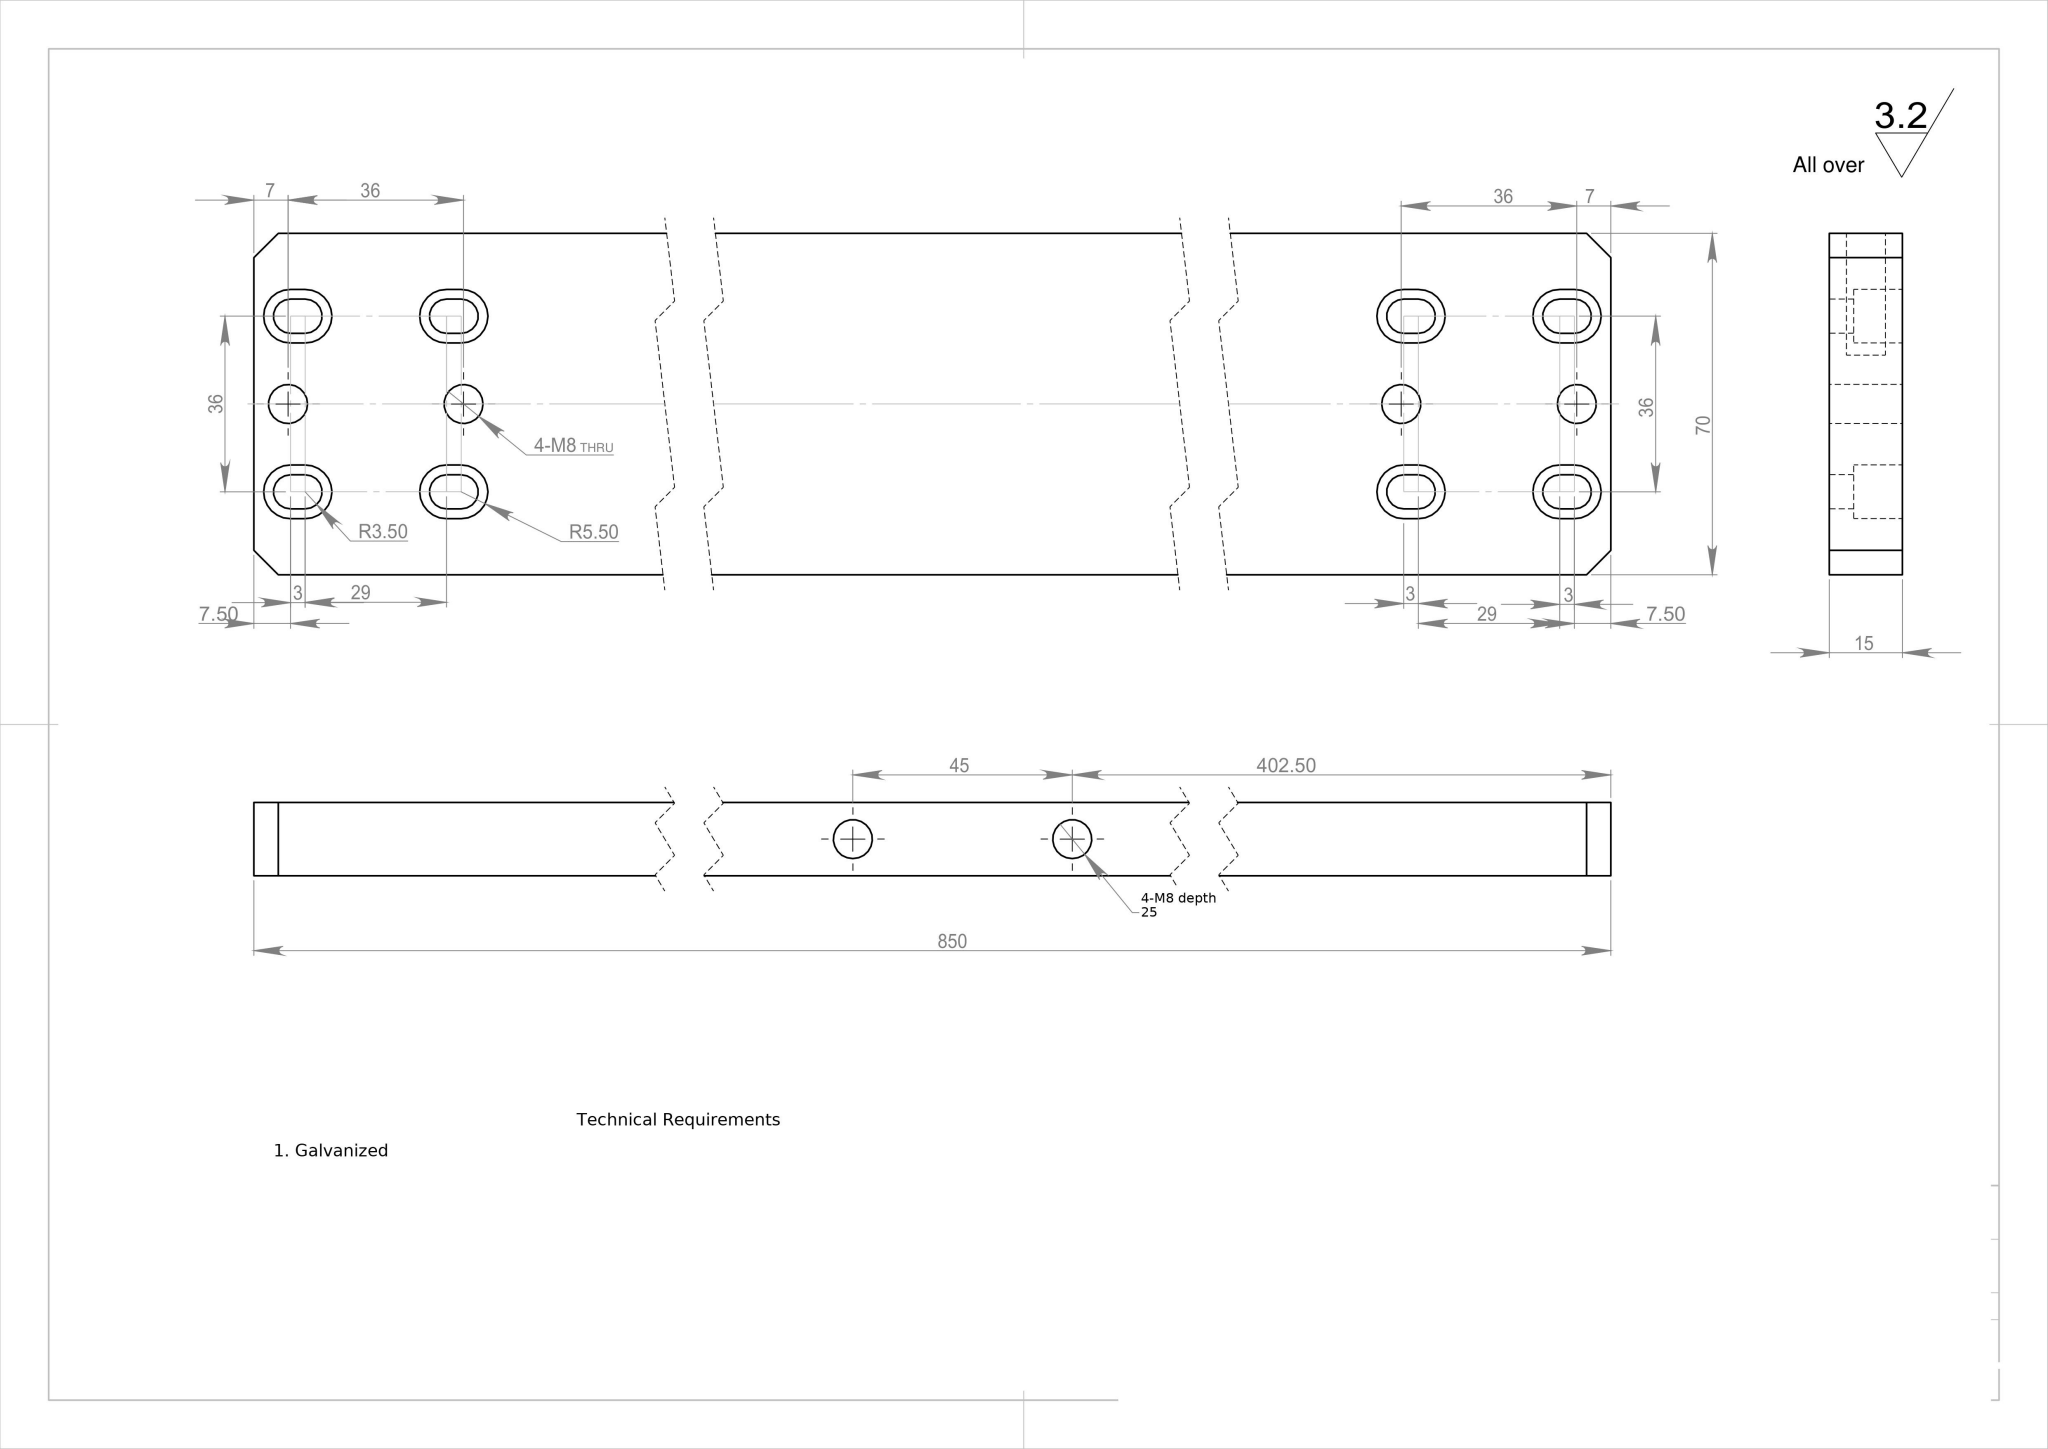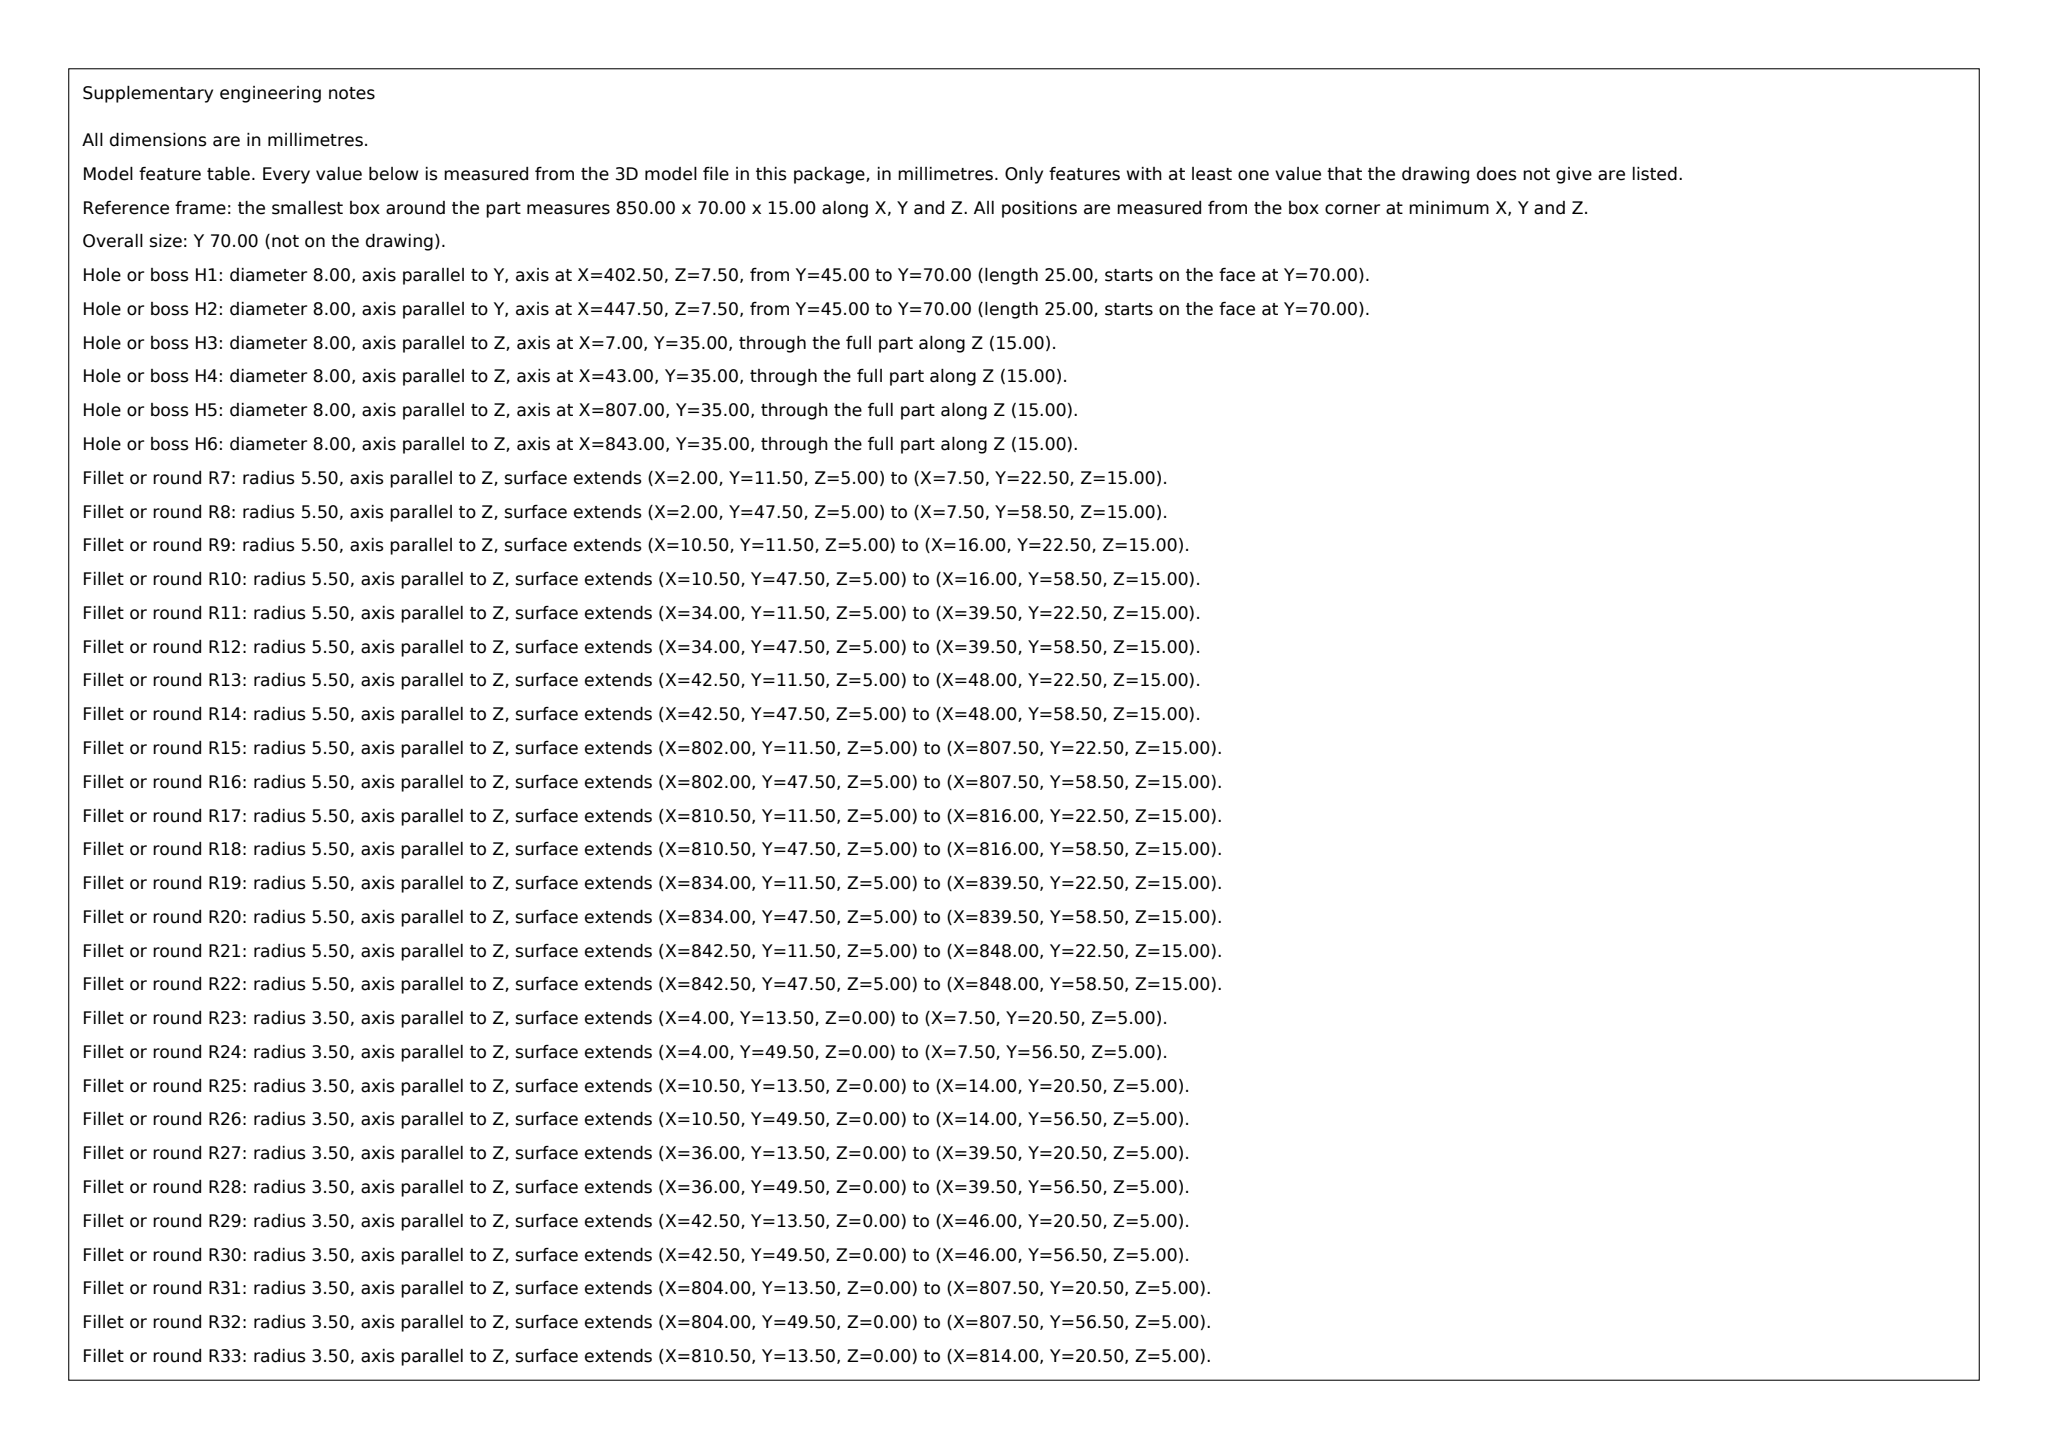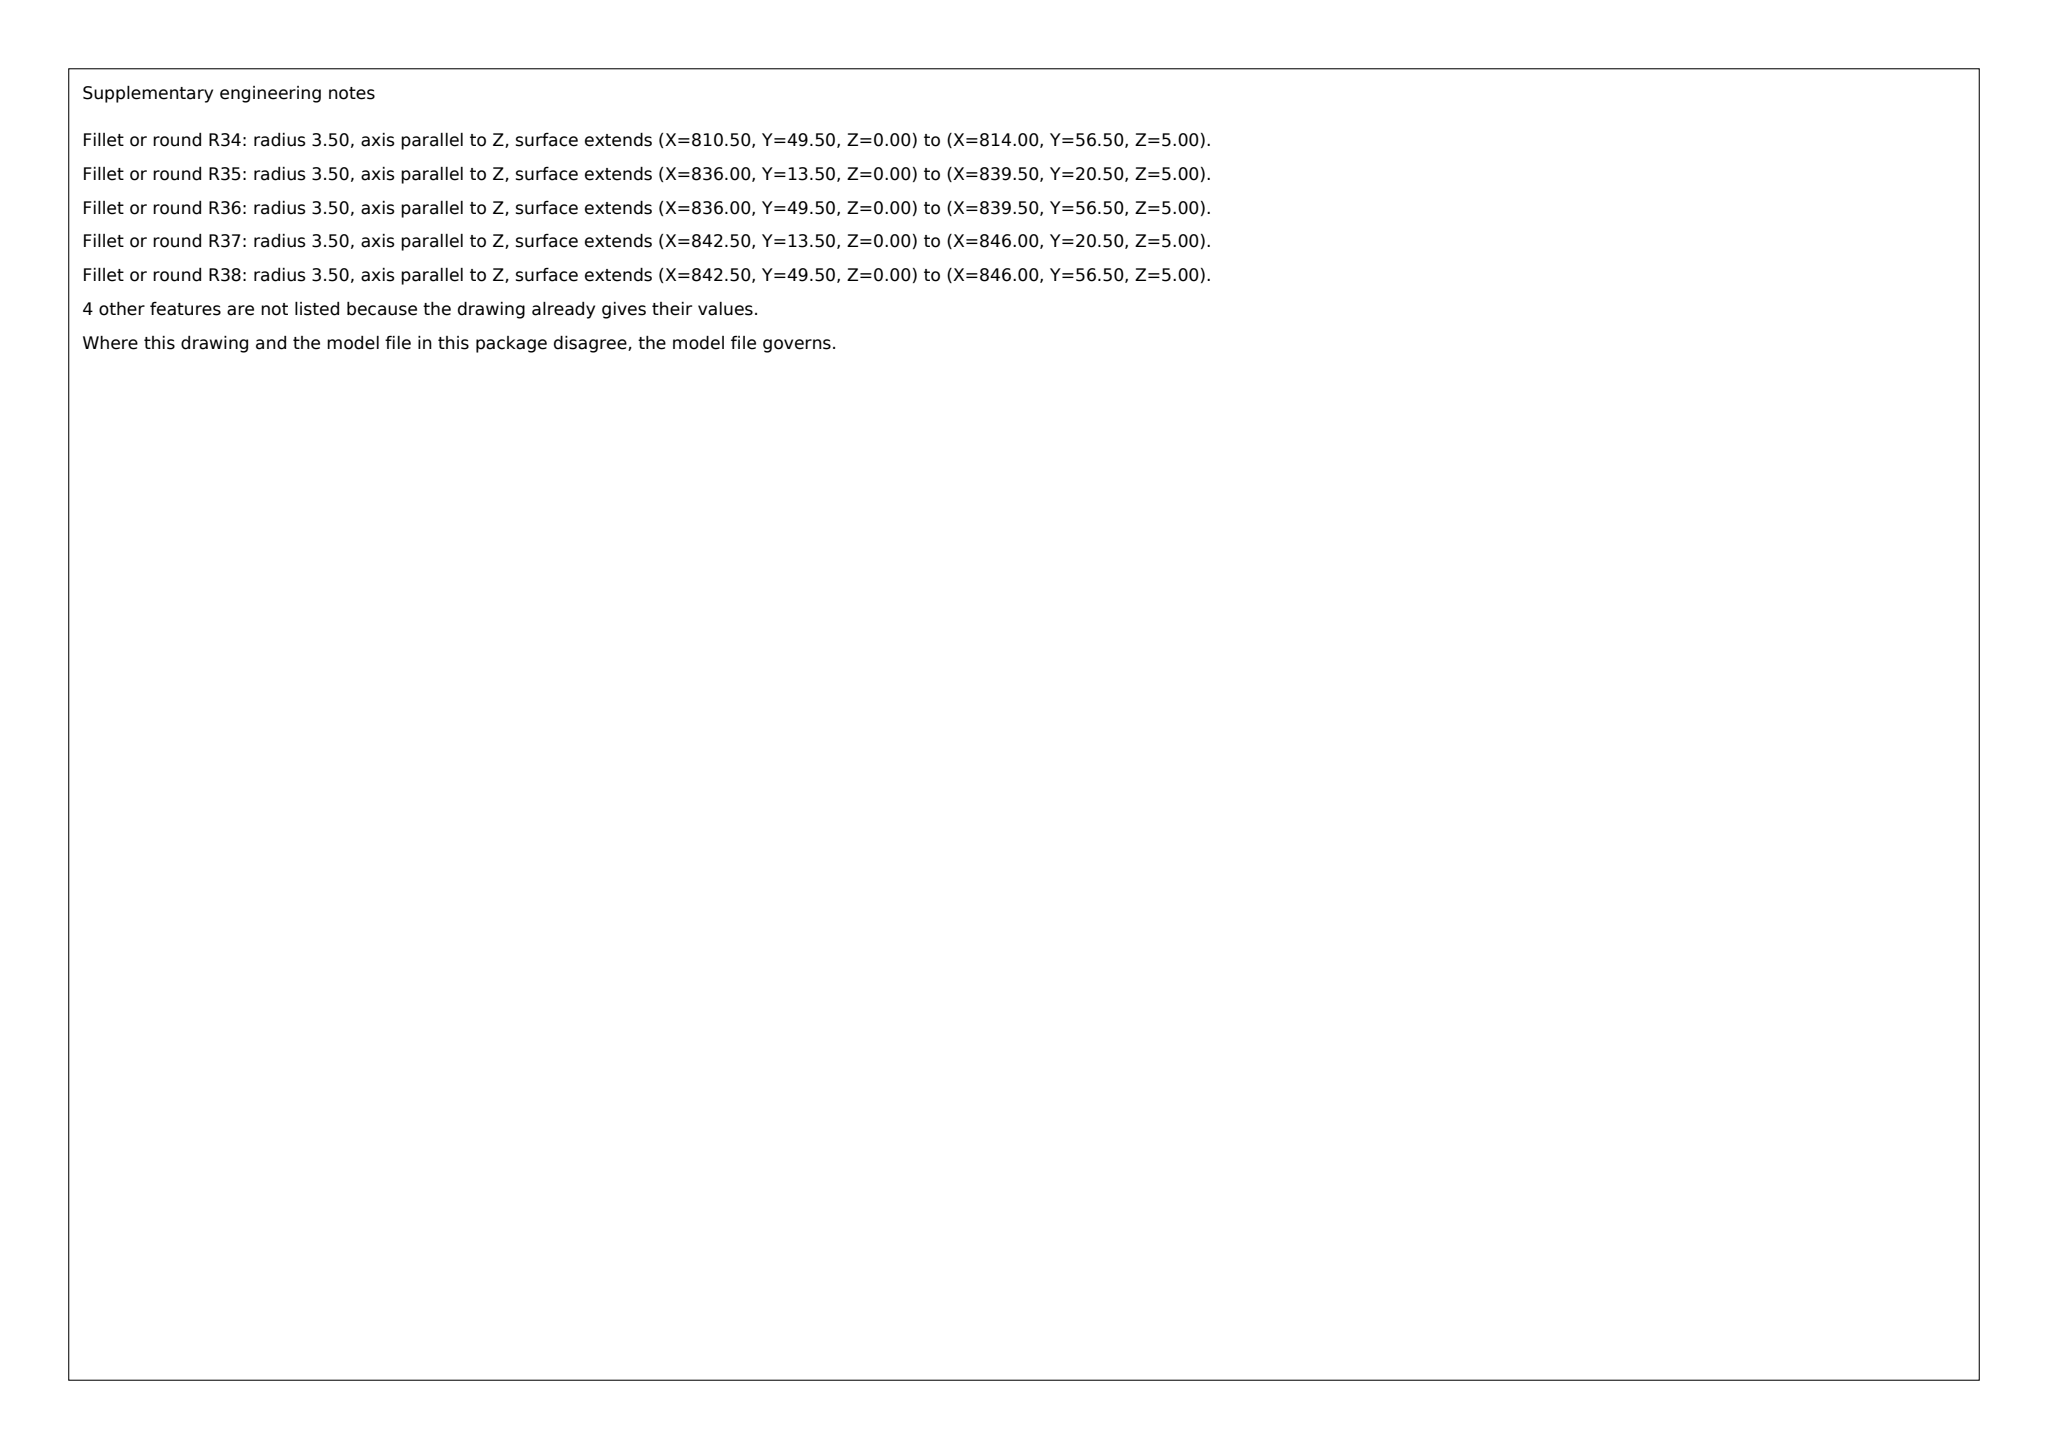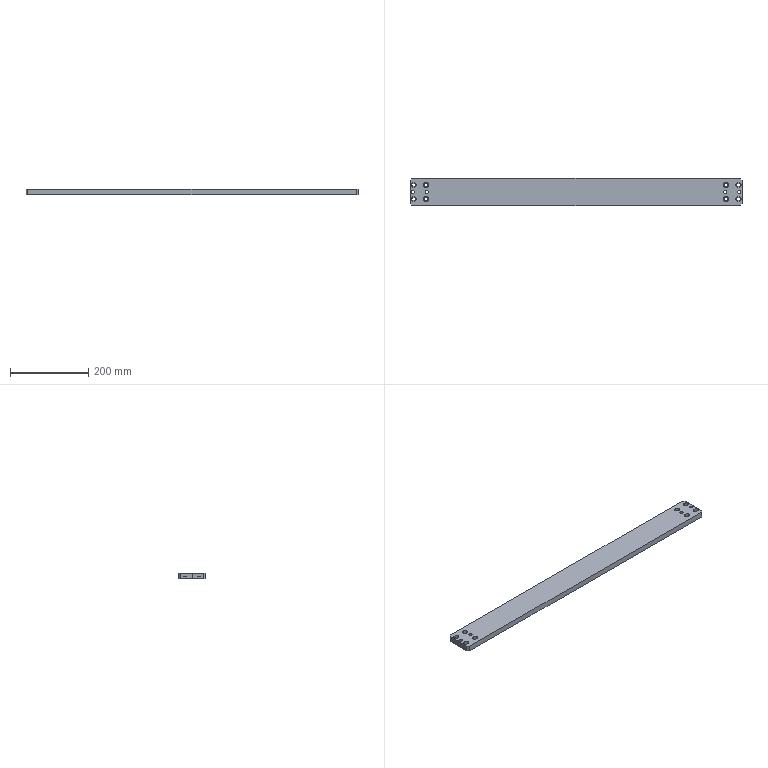Part | SolidWorks | mm | 1 solid | 112 faces | box 850 x 70 x 15 mm | volume 873599 mm3 | cylinder 60 | plane 52 | commonest cylinder face diameters 11 x24 7 x24 8 x12
build123d program:
from build123d import *

# Parameters (mm, degrees)
SKETCH1_W            = 850
SKETCH1_H            = 70
BOSS_EXTRUDE1_DEPTH  = 15
CUT_EXTRUDE1_DEPTH   = 427.702
CUT_EXTRUDE2_DEPTH   = 10
LPATTERN1_COUNT      = 2
LPATTERN1_PITCH      = 32
MIRROR1_COPY_1_DEPTH = 427.702
MIRROR1_COPY_2_DEPTH = 10
MIRROR2_COPY_1_DEPTH = 427.702
MIRROR2_COPY_2_DEPTH = 10
MIRROR2_COPY_3_DEPTH = 427.702
MIRROR2_COPY_4_DEPTH = 10
MIRROR2_COPY_5_DEPTH = 427.702
MIRROR2_COPY_6_DEPTH = 10
CHAMFER1_SIZE        = 5
SKETCH5_R            = 4
CUT_EXTRUDE4_DEPTH   = 25
SKETCH7_R            = 4
CUT_EXTRUDE5_DEPTH   = 427.702


with BuildPart() as part:
    # Sketch1 → Boss-Extrude1 (new body)
    with BuildSketch(Plane.XY):
        Rectangle(SKETCH1_W, SKETCH1_H)
    extrude(amount=BOSS_EXTRUDE1_DEPTH)

    # Sketch2 → Cut-Extrude1 (cut, through all)
    with BuildSketch(Plane.XY.offset(15)):
        with BuildLine():
            Line((-417.5, 21.5), (-414.5, 21.5))
            ThreePointArc((-414.5, 21.5), (-411, 18), (-414.5, 14.5))
            Line((-414.5, 14.5), (-417.5, 14.5))
            ThreePointArc((-417.5, 14.5), (-421, 18), (-417.5, 21.5))
        make_face()
    cut_extrude1 = extrude(amount=-CUT_EXTRUDE1_DEPTH, mode=Mode.SUBTRACT)

    # Sketch3 → Cut-Extrude2 (cut)
    with BuildSketch(Plane.XY.offset(15)):
        with BuildLine():
            Line((-417.5, 12.5), (-414.5, 12.5))
            ThreePointArc((-414.5, 12.5), (-409, 18), (-414.5, 23.5))
            Line((-414.5, 23.5), (-417.5, 23.5))
            ThreePointArc((-417.5, 23.5), (-423, 18), (-417.5, 12.5))
        make_face()
    cut_extrude2 = extrude(amount=-CUT_EXTRUDE2_DEPTH, mode=Mode.SUBTRACT)

    # LPattern1: Cut-Extrude1, Cut-Extrude2 ×2
    with Locations(*[(i * LPATTERN1_PITCH, 0, 0) for i in range(1, LPATTERN1_COUNT)]):
        add(cut_extrude1, mode=Mode.SUBTRACT)
        add(cut_extrude2, mode=Mode.SUBTRACT)

    # Mirror1: Cut-Extrude1, Cut-Extrude2 across plane
    add(cut_extrude1.mirror(Plane.ZX), mode=Mode.SUBTRACT)
    add(cut_extrude2.mirror(Plane.ZX), mode=Mode.SUBTRACT)

    # Mirror1 copy 1 sketch → Mirror1 copy 1 (cut, through all)
    with BuildSketch(Plane(origin=(32, 0, 15), x_dir=(1, 0, 0), z_dir=(0, 0, 1))):
        with BuildLine():
            Line((-417.5, -21.5), (-414.5, -21.5))
            ThreePointArc((-414.5, -21.5), (-411, -18), (-414.5, -14.5))
            Line((-414.5, -14.5), (-417.5, -14.5))
            ThreePointArc((-417.5, -14.5), (-421, -18), (-417.5, -21.5))
        make_face()
    extrude(amount=-MIRROR1_COPY_1_DEPTH, mode=Mode.SUBTRACT)

    # Mirror1 copy 2 sketch → Mirror1 copy 2 (cut)
    with BuildSketch(Plane(origin=(32, 0, 15), x_dir=(1, 0, 0), z_dir=(0, 0, 1))):
        with BuildLine():
            Line((-417.5, -12.5), (-414.5, -12.5))
            ThreePointArc((-414.5, -12.5), (-409, -18), (-414.5, -23.5))
            Line((-414.5, -23.5), (-417.5, -23.5))
            ThreePointArc((-417.5, -23.5), (-423, -18), (-417.5, -12.5))
        make_face()
    extrude(amount=-MIRROR1_COPY_2_DEPTH, mode=Mode.SUBTRACT)

    # Mirror2: Cut-Extrude1, Cut-Extrude2 across plane
    add(cut_extrude1.mirror(Plane(origin=(0, 0, 0), x_dir=(0, 0, 1), z_dir=(1, 0, 0))), mode=Mode.SUBTRACT)
    add(cut_extrude2.mirror(Plane(origin=(0, 0, 0), x_dir=(0, 0, 1), z_dir=(1, 0, 0))), mode=Mode.SUBTRACT)

    # Mirror2 copy 1 sketch → Mirror2 copy 1 (cut, through all)
    with BuildSketch(Plane(origin=(-32, 0, 15), x_dir=(-1, 0, 0), z_dir=(0, 0, 1))):
        with BuildLine():
            Line((-417.5, -21.5), (-414.5, -21.5))
            ThreePointArc((-414.5, -21.5), (-411, -18), (-414.5, -14.5))
            Line((-414.5, -14.5), (-417.5, -14.5))
            ThreePointArc((-417.5, -14.5), (-421, -18), (-417.5, -21.5))
        make_face()
    extrude(amount=-MIRROR2_COPY_1_DEPTH, mode=Mode.SUBTRACT)

    # Mirror2 copy 2 sketch → Mirror2 copy 2 (cut)
    with BuildSketch(Plane(origin=(-32, 0, 15), x_dir=(-1, 0, 0), z_dir=(0, 0, 1))):
        with BuildLine():
            Line((-417.5, -12.5), (-414.5, -12.5))
            ThreePointArc((-414.5, -12.5), (-409, -18), (-414.5, -23.5))
            Line((-414.5, -23.5), (-417.5, -23.5))
            ThreePointArc((-417.5, -23.5), (-423, -18), (-417.5, -12.5))
        make_face()
    extrude(amount=-MIRROR2_COPY_2_DEPTH, mode=Mode.SUBTRACT)

    # Mirror2 copy 3 sketch → Mirror2 copy 3 (cut, through all)
    with BuildSketch(Plane(origin=(0, 0, 15), x_dir=(-1, 0, 0), z_dir=(0, 0, 1))):
        with BuildLine():
            Line((-417.5, 21.5), (-414.5, 21.5))
            ThreePointArc((-414.5, 21.5), (-411, 18), (-414.5, 14.5))
            Line((-414.5, 14.5), (-417.5, 14.5))
            ThreePointArc((-417.5, 14.5), (-421, 18), (-417.5, 21.5))
        make_face()
    extrude(amount=-MIRROR2_COPY_3_DEPTH, mode=Mode.SUBTRACT)

    # Mirror2 copy 4 sketch → Mirror2 copy 4 (cut)
    with BuildSketch(Plane(origin=(0, 0, 15), x_dir=(-1, 0, 0), z_dir=(0, 0, 1))):
        with BuildLine():
            Line((-417.5, 12.5), (-414.5, 12.5))
            ThreePointArc((-414.5, 12.5), (-409, 18), (-414.5, 23.5))
            Line((-414.5, 23.5), (-417.5, 23.5))
            ThreePointArc((-417.5, 23.5), (-423, 18), (-417.5, 12.5))
        make_face()
    extrude(amount=-MIRROR2_COPY_4_DEPTH, mode=Mode.SUBTRACT)

    # Mirror2 copy 5 sketch → Mirror2 copy 5 (cut, through all)
    with BuildSketch(Plane(origin=(-32, 0, 15), x_dir=(-1, 0, 0), z_dir=(0, 0, 1))):
        with BuildLine():
            Line((-417.5, 21.5), (-414.5, 21.5))
            ThreePointArc((-414.5, 21.5), (-411, 18), (-414.5, 14.5))
            Line((-414.5, 14.5), (-417.5, 14.5))
            ThreePointArc((-417.5, 14.5), (-421, 18), (-417.5, 21.5))
        make_face()
    extrude(amount=-MIRROR2_COPY_5_DEPTH, mode=Mode.SUBTRACT)

    # Mirror2 copy 6 sketch → Mirror2 copy 6 (cut)
    with BuildSketch(Plane(origin=(-32, 0, 15), x_dir=(-1, 0, 0), z_dir=(0, 0, 1))):
        with BuildLine():
            Line((-417.5, 12.5), (-414.5, 12.5))
            ThreePointArc((-414.5, 12.5), (-409, 18), (-414.5, 23.5))
            Line((-414.5, 23.5), (-417.5, 23.5))
            ThreePointArc((-417.5, 23.5), (-423, 18), (-417.5, 12.5))
        make_face()
    extrude(amount=-MIRROR2_COPY_6_DEPTH, mode=Mode.SUBTRACT)

    # Chamfer1
    chamfer1_edges = [part.edges().sort_by_distance(p)[0] for p in [
        (425, -35, 7.5),
        (-425, -35, 7.5),
        (-425, 35, 7.5),
        (425, 35, 7.5),
    ]]
    chamfer(chamfer1_edges, length=CHAMFER1_SIZE)

    # Sketch5 → Cut-Extrude4 (cut)
    with BuildSketch(Plane(origin=(0, 35, 0), x_dir=(1, 0, 0), z_dir=(0, 1, 0))):
        with Locations(Location((-22.5, -7.5, 0), (0, 0, 270))):
            Circle(SKETCH5_R)
    cut_extrude4 = extrude(amount=-CUT_EXTRUDE4_DEPTH, mode=Mode.SUBTRACT)

    # Mirror3: Cut-Extrude4 across plane
    add(cut_extrude4.mirror(Plane(origin=(0, 0, 0), x_dir=(0, 0, 1), z_dir=(1, 0, 0))), mode=Mode.SUBTRACT)

    # Sketch7 → Cut-Extrude5 (cut, through all)
    with BuildSketch(Plane.XY.offset(15)):
        with Locations((-418, 0)):
            Circle(SKETCH7_R)
        with Locations((-382, 0)):
            Circle(SKETCH7_R)
    cut_extrude5 = extrude(amount=-CUT_EXTRUDE5_DEPTH, mode=Mode.SUBTRACT)

    # Mirror4: Cut-Extrude5 across plane
    add(cut_extrude5.mirror(Plane(origin=(0, 0, 0), x_dir=(0, 0, 1), z_dir=(1, 0, 0))), mode=Mode.SUBTRACT)


solid = part.part